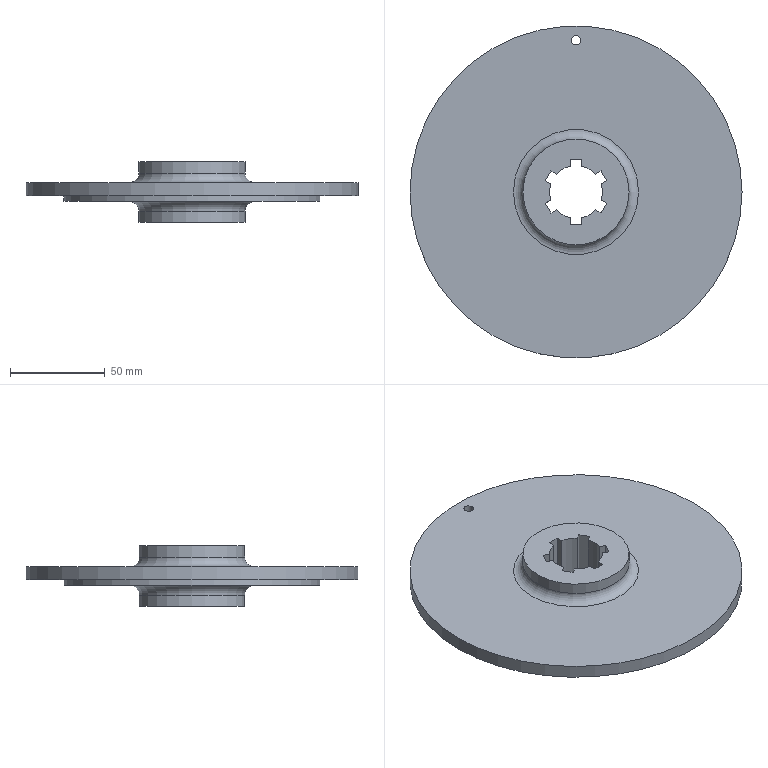Component | NX | CLUTCH_PLATE | 1 solid | 36 faces | volume 244099 mm3 | plane 23 | cylinder 11 | torus 2 | commonest cylinder face diameters 28 x6 56 x2 135 x1 175 x1 5 x1